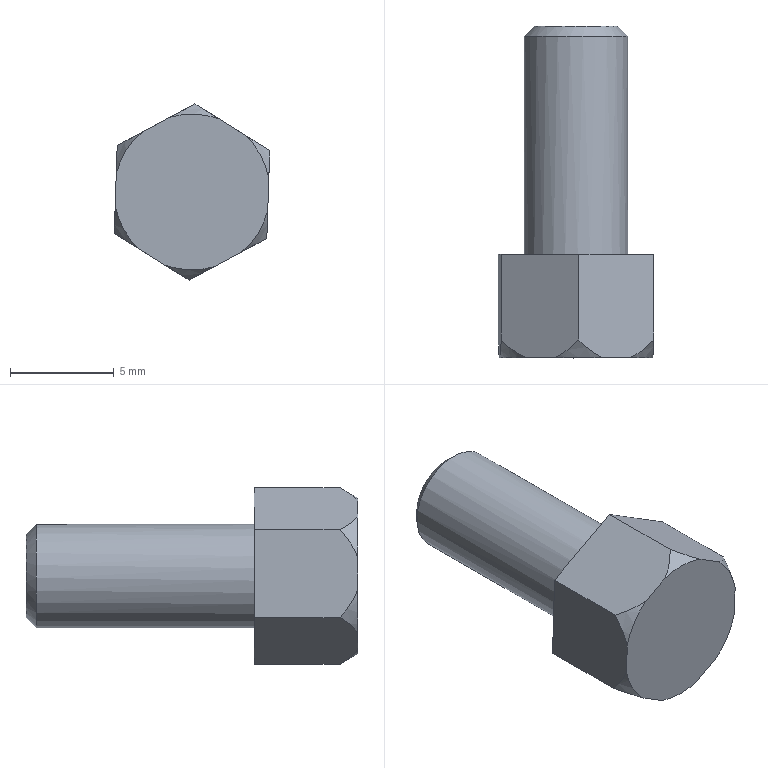Component | NX | HEX_SCREW | 1 solid | 17 faces | volume 448 mm3 | plane 9 | cone 7 | cylinder 1 | commonest cylinder face diameters 5 x1